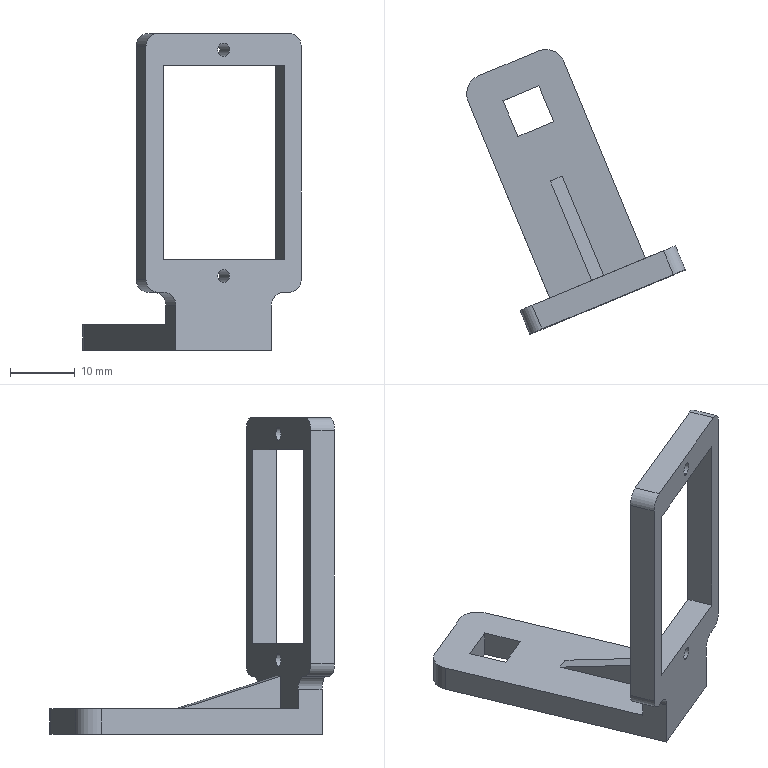Component | SolidWorks | SteeringPlate-1 | 1 solid | 35 faces | box 33.8 x 44.07 x 49 mm | volume 4483 mm3 | plane 23 | cylinder 12 | commonest cylinder face diameters 4 x6 2 x4 6 x2
build123d program:
from build123d import *

# Parameters (mm, degrees)
SKETCH1_2_W                  = 6
SKETCH1_2_H                  = 6
BOSS_EXTRUDE1_DEPTH          = 4
SKETCH2_R                    = 1
BOSS_EXTRUDE2_DEPTH          = 4
RIB1_REACH                   = 61.845
SKETCH4_WALL_W               = 139.15
SKETCH4_WALL_H               = 2
SERVOWINDOWRELIEF_DEPTH      = 62.326
SERVOWINDOWRELIEF_DEPTH_BACK = 62.326
SKETCH1_W                    = 0.48
SKETCH1_H                    = 30


with BuildPart() as part:
    # Sketch1_2 → Boss-Extrude1 (new body)
    with BuildSketch(Plane.XY):
        with BuildLine():
            Line((-13.667, -0.2476), (-13.667, -13.248))
            Line((-13.667, -13.248), (-13.667, -37.248))
            Line((-13.667, -37.248), (2.333, -37.248))
            Line((2.333, -37.248), (2.333, -13.248))
            Line((2.333, -13.248), (2.333, -0.2476))
            ThreePointArc((2.333, -0.2476), (1.454, 1.874), (-0.667, 2.752))
            Line((-0.667, 2.752), (-10.667, 2.752))
            ThreePointArc((-10.667, 2.752), (-12.788, 1.874), (-13.667, -0.2476))
        make_face()
        with Locations((-5.667, -5.248)):
            Rectangle(SKETCH1_2_W, SKETCH1_2_H, mode=Mode.SUBTRACT)
    extrude(amount=BOSS_EXTRUDE1_DEPTH)

    # Sketch2 → Boss-Extrude2 (add)
    with BuildSketch(Plane.XZ.offset(37.248)):
        with BuildLine():
            Line((-13.667, 0), (2.333, 0))
            Line((2.333, 0), (2.333, -3))
            ThreePointArc((2.333, -3), (2.919, -4.414), (4.333, -5))
            Line((4.333, -5), (5.333, -5))
            ThreePointArc((5.333, -5), (6.747, -5.586), (7.333, -7))
            Line((7.333, -7), (7.333, -43))
            ThreePointArc((7.333, -43), (6.747, -44.414), (5.333, -45))
            Line((5.333, -45), (-16.667, -45))
            ThreePointArc((-16.667, -45), (-18.081, -44.414), (-18.667, -43))
            Line((-18.667, -43), (-18.667, -7))
            ThreePointArc((-18.667, -7), (-18.081, -5.586), (-16.667, -5))
            Line((-16.667, -5), (-15.667, -5))
            ThreePointArc((-15.667, -5), (-14.253, -4.414), (-13.667, -3))
            Line((-13.667, -3), (-13.667, 0))
        make_face()
        with Locations(Location((-5.667, -42.5, 0), (0, 0, 270))):
            Circle(SKETCH2_R, mode=Mode.SUBTRACT)
        with Locations(Location((-5.667, -7.5, 0), (0, 0, 270))):
            Circle(SKETCH2_R, mode=Mode.SUBTRACT)
        Polygon((-13.667, -40), (2.333, -40), (4.155, -40), (4.155, -10), (2.333, -10), (-2.667, -10), (-8.667, -10), (-13.667, -10), (-15.933, -10), (-15.933, -40), align=None, mode=Mode.SUBTRACT)
    extrude(amount=-BOSS_EXTRUDE2_DEPTH)

    # Sketch4 wall → Rib1 (add, up to next)
    with BuildSketch(Plane(origin=(-5.67, -24.884, -2.5), x_dir=(0, -0.9581, -0.2864), z_dir=(0, 0.2864, -0.9581)), mode=Mode.PRIVATE) as rib1_sk1:
        Rectangle(SKETCH4_WALL_W, SKETCH4_WALL_H)
    rib1_tool1 = extrude(rib1_sk1.sketch, amount=-RIB1_REACH, mode=Mode.PRIVATE) - part.part
    add(rib1_tool1.solids().sort_by_distance((-5.67, -24.884, -2.5))[0])

    # Sketch1 → ServoWindowRelief (cut, two sides: drawn at the far end of the back side and taken through both)
    with BuildSketch(Plane(origin=(0, 0, 0), x_dir=(1, 0, 0), z_dir=(0, 1, 0)).offset(-SERVOWINDOWRELIEF_DEPTH_BACK)):
        with Locations((4.24, 25)):
            Rectangle(SKETCH1_W, SKETCH1_H)
    extrude(amount=SERVOWINDOWRELIEF_DEPTH + SERVOWINDOWRELIEF_DEPTH_BACK, mode=Mode.SUBTRACT)


solid = part.part

# Placed as in the assembly
solid = solid.moved(Location((12.906, 35.602, 387.846), (180, 0, 157.477)))